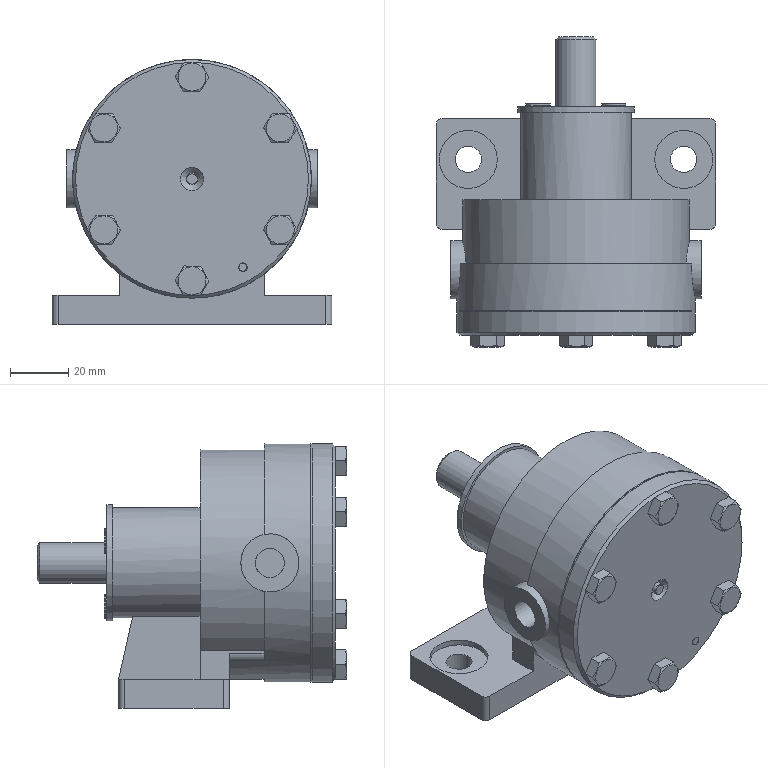Assembly | NX | mm | 20 component files | 20 solids | 361 faces | box 96 x 106.5 x 91 mm | volume 286159 mm3 | plane 173 | cylinder 103 | spline 48 | cone 37 | commonest cylinder face diameters 6 x16 4 x12 7 x12 5 x9 8.4 x6 8 x6 48 x4 20 x4
Bill of materials:
unnamed part 1 | 1 |  | Rectangular block with one round hole passing through it between two opposite side faces.
unnamed part 2 | 1 |  | Very thin flat ring with a large central opening, six evenly spaced holes on a circle, and one smaller hole set off between two of them.
unnamed part 3 | 6 |  | Hex-head bolt shape with a threaded shank that appears to be threaded along its full length.
unnamed part 4 | 1 |  | Short cylindrical sleeve with two opposite rectangular windows cut through the wall at mid-height. This leaves two end rings joined by two axial bridges.
unnamed part 5 | 1 |  | U-shaped (C-channel) piece with a flat web and two parallel flanges. The flange ends are curved (arched) in plan view, and the edges are lightly chamfered.
unnamed part 6 | 1 |  | Plain thick flat ring (washer-like annulus) with a rectangular cross-section.
unnamed part 7 | 1 |  | Circular disc or plate with a chamfered outer edge and a shallow raised circular boss on one face. It has six evenly spaced through-holes on a circle, one smaller offset hole, and a small central hole with a countersink or counterbore.
unnamed part 8 | 3 |  | Slotted countersunk (flat-head) screw shape: a conical head with a straight slot across its top and a threaded cylindrical shank.
unnamed part 9 | 1 |  | Plain solid cylindrical pin with small chamfers at both ends.
unnamed part 10 | 1 |  | Clevis-like part: a cylindrical head with a slot cut across one end, forming two prongs with a cross hole through them. A small stepped collar sits behind the head, and a slender stepped shaft with a chamfered tip extends from it.
unnamed part 11 | 1 |  | Stepped cylindrical pin with two coaxial diameters: a larger section with a chamfered end and a smaller section with a lightly chamfered end.
unnamed part 12 | 1 |  | Thin flat circular disc with a large central hole and three smaller holes evenly spaced on a circle.
unnamed part 13 | 1 |  | Housing with a cylindrical body that is open on one end, sitting on a rectangular foot plate. The open end has a thick annular rim with a ring of small holes. A smaller cylindrical boss sticks out from the opposite end. Short cylindrical lugs with cross holes stick out from both sides. The foot plate has two mounting holes and extends to either side of the body, which is joined to it by a pedestal.
Mates:
1. fix | pump_body 1 component
2. concentric | bushing 1 arc | pump_body 1 edge
3. concentric | pump_body 1 edge | rotor_shaft 1 edge
4. concentric | large_slider 1 edge | bushing 1 edge
5. parallel | bushing 1 face | pump_body 1 face
6. parallel | rotor_shaft 1 face | large_slider 1 face
7. touch align | small_slider 1 face | large_slider 1 face
8. center | small_slider 1 face | small_slider 1 face | rotor_shaft 1 face | rotor_shaft 1 face
9. center | small_slider 1 face | small_slider 1 face | large_slider 1 face | large_slider 1 face
10. concentric | small_shaft 1 edge | small_slider 1 edge
11. concentric | seal_ring 1 arc | pump_body 1 edge
12. concentric | gland 1 arc | pump_body 1 edge
13. concentric | pump_body 1 arc | gland 1 arc
14. concentric | gasket 1 arc | pump_body 1 edge
15. concentric | gasket 1 arc | pump_body 1 edge
16. concentric | gasket 1 edge | pump_cover 1 edge
17. concentric | gasket 1 edge | pump_cover 1 edge
18. concentric | pin 1 | pump_cover 1 edge
19. touch align | bolt 6 face | pump_cover 1 face
20. touch align | pump_cover 1 face | bolt 6 face
21. fix | assembly component
22. bond | bolt 6 component | assembly component
23. bond | bolt 5 component | assembly component
24. bond | bolt 4 component | assembly component
25. bond | bolt 3 component | assembly component
26. bond | bolt 2 component | assembly component
27. circular | assembly datumaxis | assembly cartesiancoordinatesystem | assembly cartesiancoordinatesystem | assembly cartesiancoordinatesystem | assembly cartesiancoordinatesystem | assembly cartesiancoordinatesystem | assembly cartesiancoordinatesystem
28. bond | bolt 1 component | assembly component
29. touch align | screw 3 | gland 1 face
30. touch align | screw 3 | gland 1 face
31. fix | assembly component
32. bond | screw 3 component | assembly component
33. bond | screw 2 component | assembly component
34. bond | screw 1 component | assembly component
35. circular | assembly datumaxis | assembly cartesiancoordinatesystem | assembly cartesiancoordinatesystem | assembly cartesiancoordinatesystem